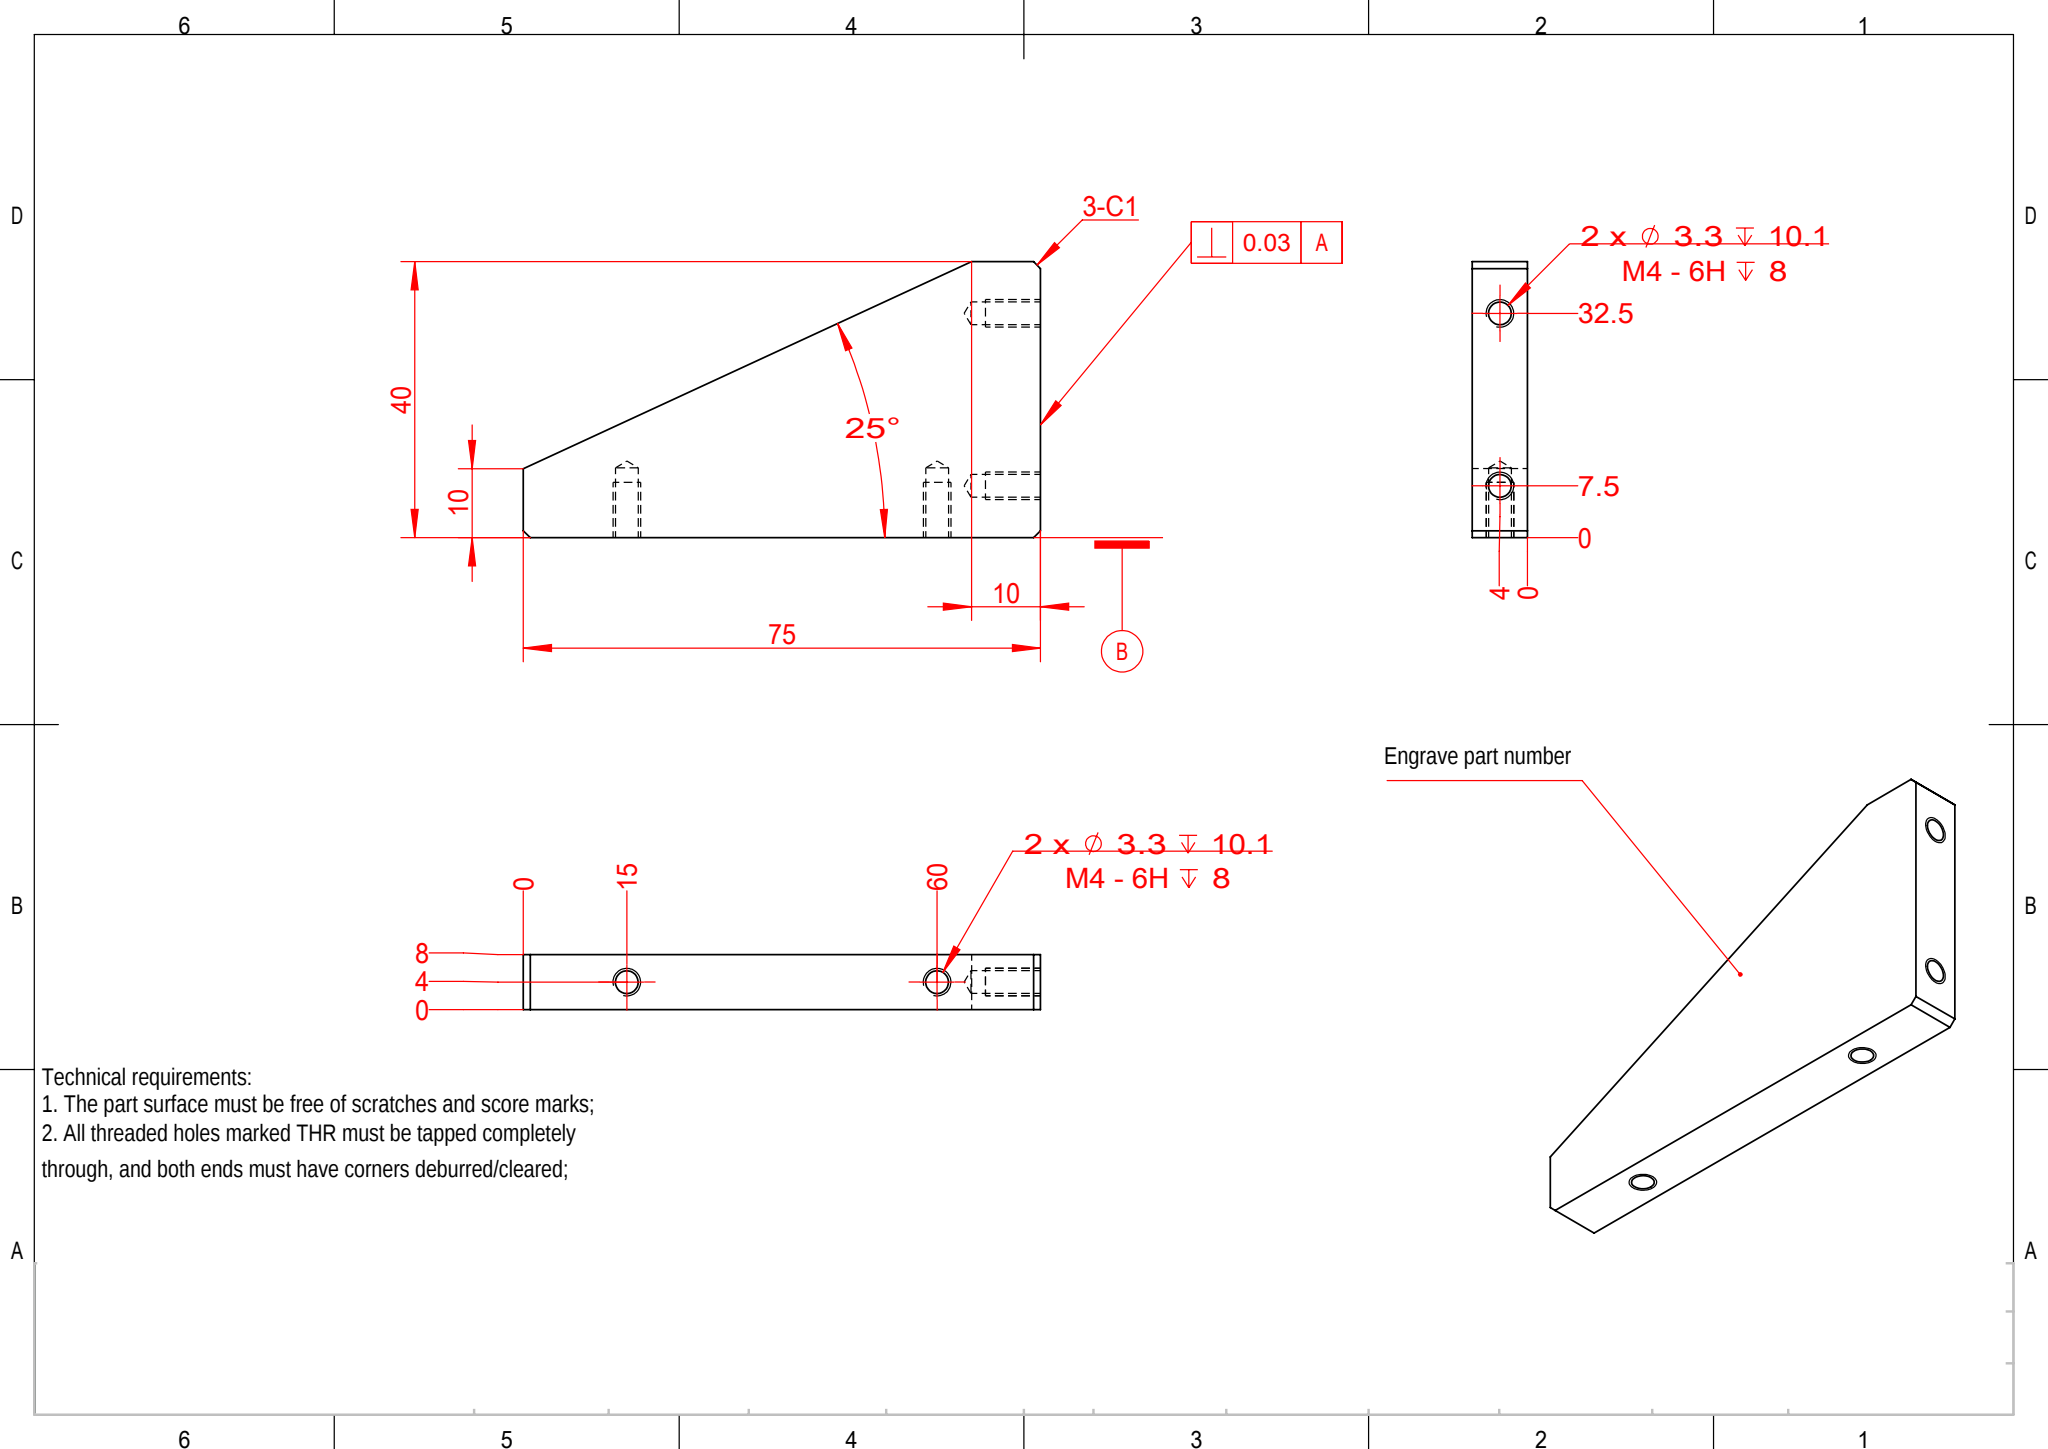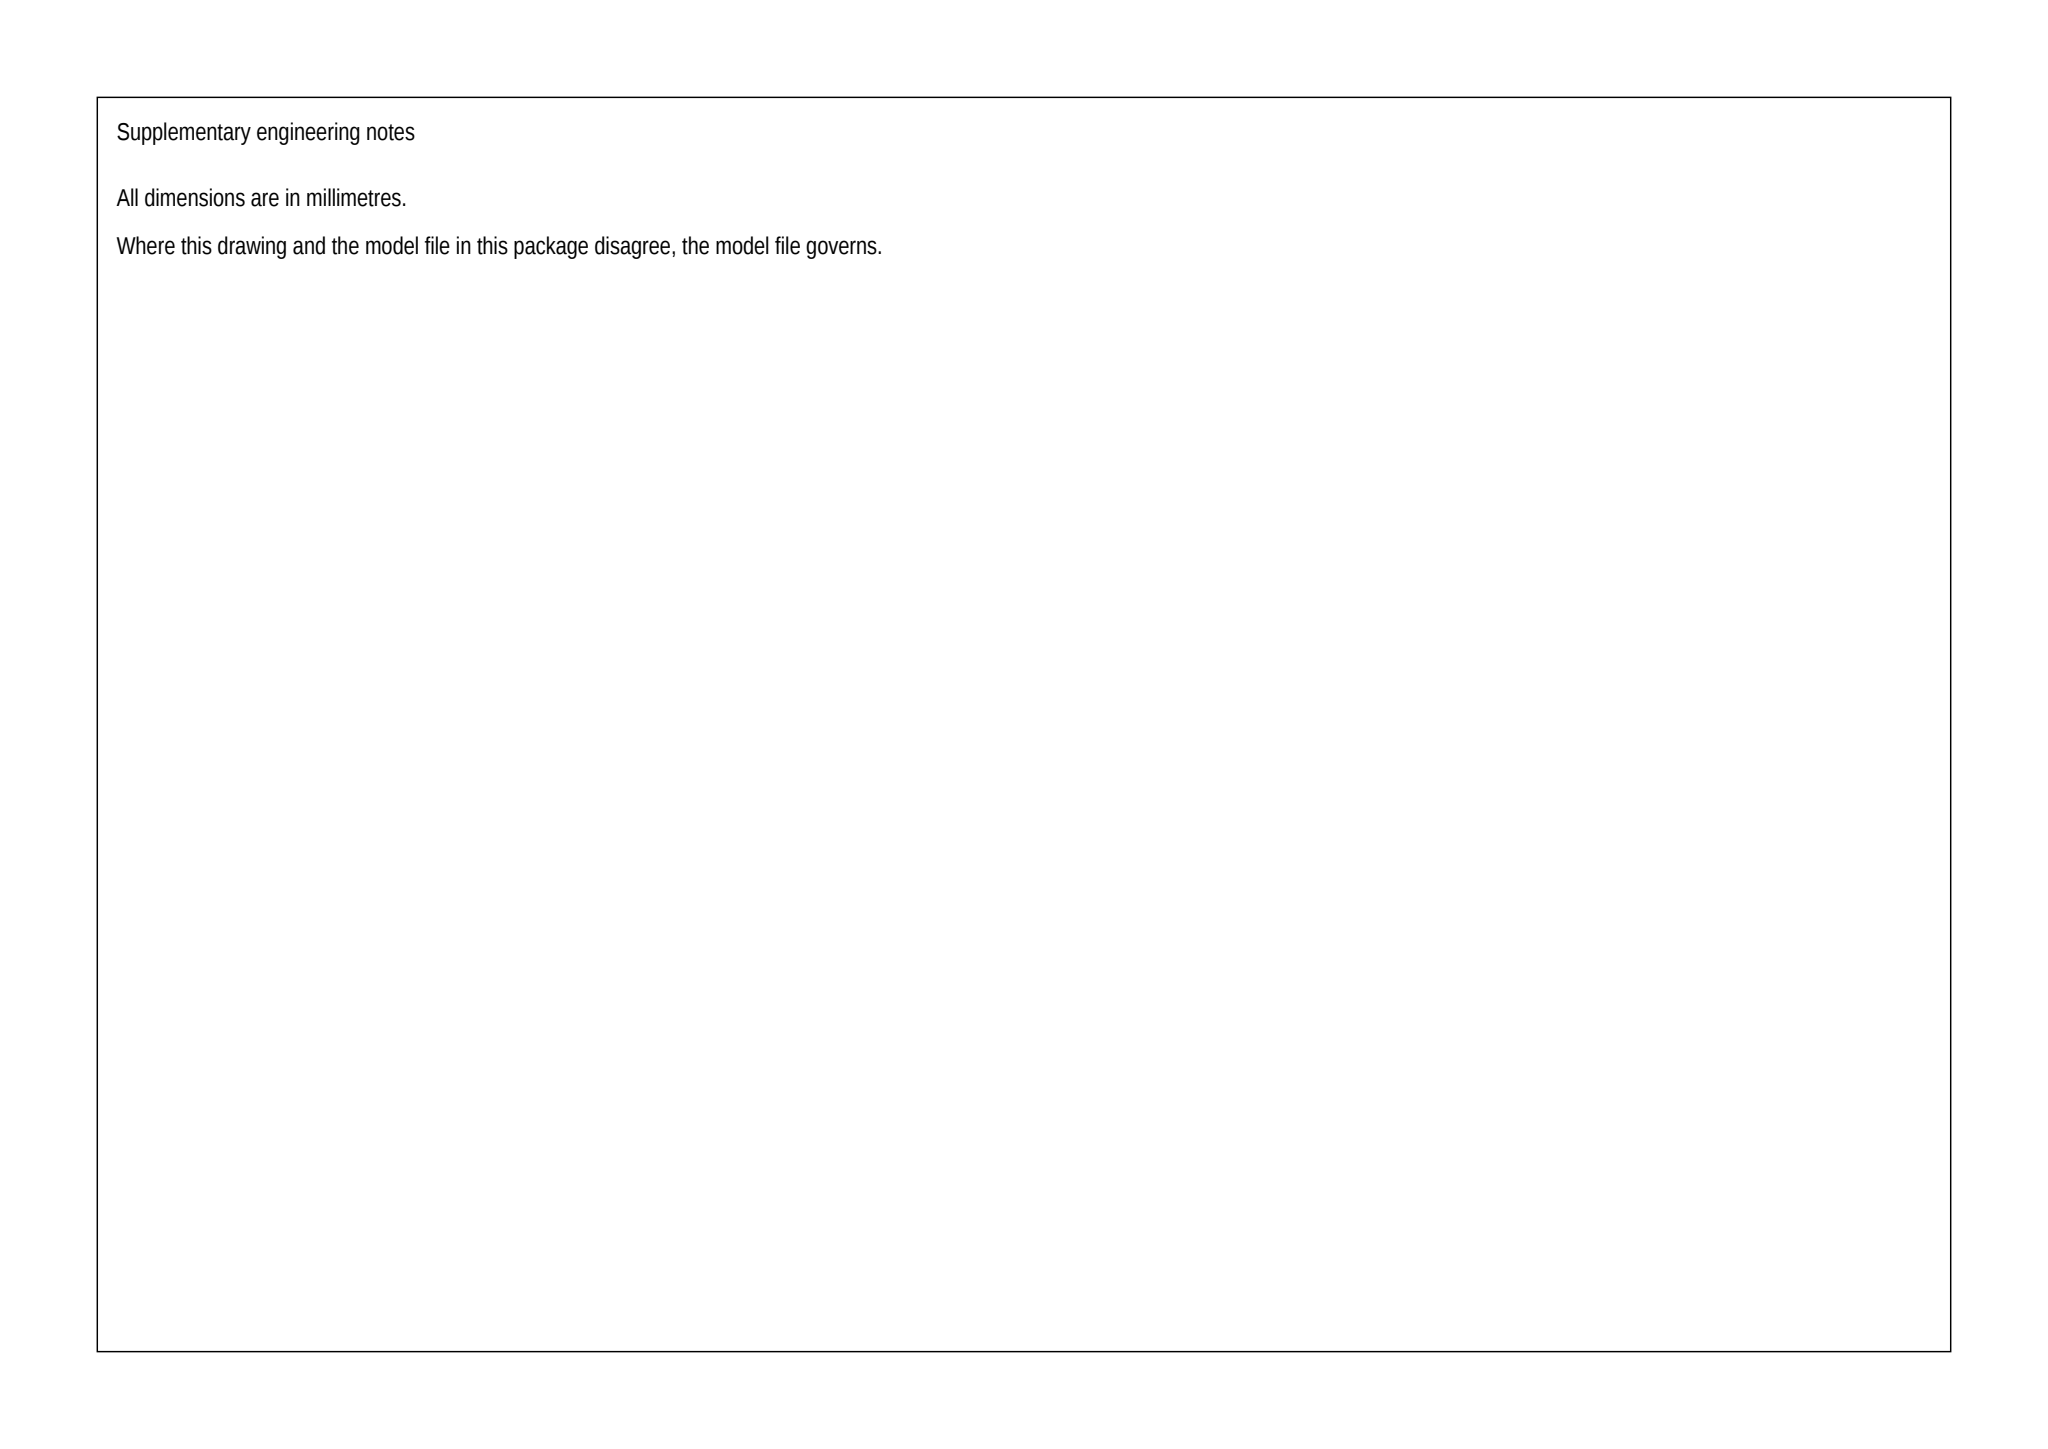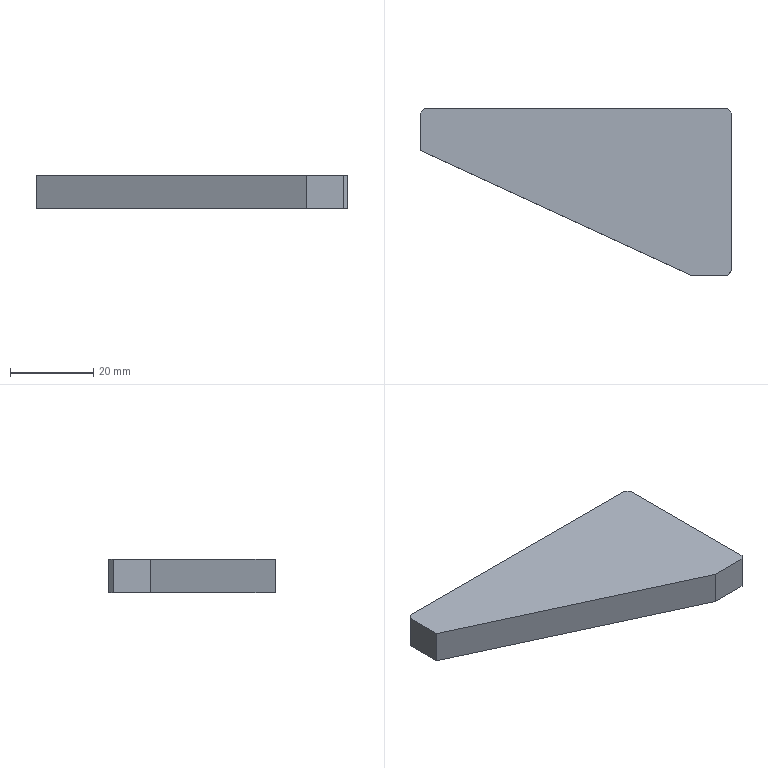Part | SolidWorks | mm | 1 solid | 26 faces | box 75 x 40 x 8 mm | volume 15831 mm3 | plane 10 | cylinder 8 | cone 8 | commonest cylinder face diameters 3.3 x8
build123d program:
from build123d import *

# Parameters (mm, degrees)
SKETCH1_W             = 75
SKETCH1_H             = 40
BOSS_EXTRUDE1_DEPTH   = 8
CUT_EXTRUDE1_DEPTH    = 44.246
M4_TAPPED_HOLE1_D     = 3.3
M4_TAPPED_HOLE1_DEPTH = 10.1
M4_TAPPED_HOLE1_TIP   = 0.9914
M4_TAPPED_HOLE2_D     = 3.3
M4_TAPPED_HOLE2_DEPTH = 10.1
M4_TAPPED_HOLE2_TIP   = 0.9914
CHAMFER1_SIZE         = 1


with BuildPart() as part:
    # Sketch1 → Boss-Extrude1 (new body)
    with BuildSketch(Plane.XY):
        Rectangle(SKETCH1_W, SKETCH1_H)
    extrude(amount=BOSS_EXTRUDE1_DEPTH)

    # Sketch2 → Cut-Extrude1 (cut, through all)
    with BuildSketch(Plane.XY.offset(8)):
        Polygon((-37.5, -20), (-37.5, 10), (27.5, -20), align=None)
    extrude(amount=-CUT_EXTRUDE1_DEPTH, mode=Mode.SUBTRACT)

    # M4 Tapped Hole1
    with Locations(Plane(origin=(0, 20, 0), x_dir=(1, 0, 0), z_dir=(0, 1, 0))):
        with Locations((22.5, -4), (-22.5, -4)):
            Hole(M4_TAPPED_HOLE1_D / 2, depth=M4_TAPPED_HOLE1_DEPTH)
            with Locations((0, 0, -(M4_TAPPED_HOLE1_DEPTH + M4_TAPPED_HOLE1_TIP / 2))):  # 118° drill point
                Cone(0, M4_TAPPED_HOLE1_D / 2, M4_TAPPED_HOLE1_TIP, mode=Mode.SUBTRACT)

    # M4 Tapped Hole2
    with Locations(Plane(origin=(37.5, 0, 0), x_dir=(0, 0, -1), z_dir=(1, 0, 0))):
        with Locations((-4, -12.5), (-4, 12.5)):
            Hole(M4_TAPPED_HOLE2_D / 2, depth=M4_TAPPED_HOLE2_DEPTH)
            with Locations((0, 0, -(M4_TAPPED_HOLE2_DEPTH + M4_TAPPED_HOLE2_TIP / 2))):  # 118° drill point
                Cone(0, M4_TAPPED_HOLE2_D / 2, M4_TAPPED_HOLE2_TIP, mode=Mode.SUBTRACT)

    # Chamfer1
    chamfer1_edges = [part.edges().sort_by_distance(p)[0] for p in [
        (37.5, -20, 4),
        (-37.5, 20, 4),
        (37.5, 20, 4),
    ]]
    chamfer(chamfer1_edges, length=CHAMFER1_SIZE)


solid = part.part
STEP:
#1=CARTESIAN_POINT('',(27.4,-12.5,5.65));
#2=VERTEX_POINT('',#1);
#3=CARTESIAN_POINT('',(27.4,-12.5,2.35));
#4=VERTEX_POINT('',#3);
#5=CARTESIAN_POINT('',(27.4,-12.5,4.));
#6=DIRECTION('',(1.,0.,0.));
#7=DIRECTION('',(0.,0.,-1.));
#8=AXIS2_PLACEMENT_3D('',#5,#6,#7);
#9=CIRCLE('',#8,1.65);
#10=EDGE_CURVE('',#2,#4,#9,.T.);
#11=ORIENTED_EDGE('',*,*,#10,.F.);
#12=CARTESIAN_POINT('',(37.5,-12.5,5.65));
#13=VERTEX_POINT('',#12);
#14=CARTESIAN_POINT('',(37.5,-12.5,5.65));
#15=DIRECTION('',(1.,0.,0.));
#16=VECTOR('',#15,1000.);
#17=LINE('',#14,#16);
#18=EDGE_CURVE('',#2,#13,#17,.T.);
#19=ORIENTED_EDGE('',*,*,#18,.T.);
#20=CARTESIAN_POINT('',(37.5,-12.5,2.35));
#21=VERTEX_POINT('',#20);
#22=CARTESIAN_POINT('',(37.5,-12.5,4.));
#23=DIRECTION('',(1.,0.,0.));
#24=DIRECTION('',(0.,0.,-1.));
#25=AXIS2_PLACEMENT_3D('',#22,#23,#24);
#26=CIRCLE('',#25,1.65);
#27=EDGE_CURVE('',#13,#21,#26,.T.);
#28=ORIENTED_EDGE('',*,*,#27,.T.);
#29=CARTESIAN_POINT('',(37.5,-12.5,2.35));
#30=DIRECTION('',(1.,0.,0.));
#31=VECTOR('',#30,1000.);
#32=LINE('',#29,#31);
#33=EDGE_CURVE('',#4,#21,#32,.T.);
#34=ORIENTED_EDGE('',*,*,#33,.F.);
#35=EDGE_LOOP('',(#11,#19,#28,#34));
#36=FACE_OUTER_BOUND('',#35,.T.);
#37=CARTESIAN_POINT('',(37.5,-12.5,4.));
#38=DIRECTION('',(1.,0.,0.));
#39=DIRECTION('',(0.,0.,-1.));
#40=AXIS2_PLACEMENT_3D('',#37,#38,#39);
#41=CYLINDRICAL_SURFACE('',#40,1.65);
#42=ADVANCED_FACE('',(#36),#41,.F.);
#43=CARTESIAN_POINT('',(26.409,-12.5,4.));
#44=VERTEX_POINT('',#43);
#45=CARTESIAN_POINT('',(27.4,-12.5,2.35));
#46=DIRECTION('',(0.515,0.,-0.8572));
#47=VECTOR('',#46,1000.);
#48=LINE('',#45,#47);
#49=EDGE_CURVE('',#44,#4,#48,.T.);
#50=ORIENTED_EDGE('',*,*,#49,.F.);
#51=CARTESIAN_POINT('',(27.4,-12.5,5.65));
#52=DIRECTION('',(0.515,0.,0.8572));
#53=VECTOR('',#52,1000.);
#54=LINE('',#51,#53);
#55=EDGE_CURVE('',#44,#2,#54,.T.);
#56=ORIENTED_EDGE('',*,*,#55,.T.);
#57=ORIENTED_EDGE('',*,*,#10,.T.);
#58=EDGE_LOOP('',(#50,#56,#57));
#59=FACE_OUTER_BOUND('',#58,.T.);
#60=CARTESIAN_POINT('',(27.4,-12.5,4.));
#61=DIRECTION('',(1.,0.,0.));
#62=DIRECTION('',(0.,0.,-1.));
#63=AXIS2_PLACEMENT_3D('',#60,#61,#62);
#64=CONICAL_SURFACE('',#63,1.65,1.03);
#65=ADVANCED_FACE('',(#59),#64,.F.);
#66=CARTESIAN_POINT('',(27.4,12.5,5.65));
#67=VERTEX_POINT('',#66);
#68=CARTESIAN_POINT('',(27.4,12.5,2.35));
#69=VERTEX_POINT('',#68);
#70=CARTESIAN_POINT('',(27.4,12.5,4.));
#71=DIRECTION('',(1.,0.,0.));
#72=DIRECTION('',(0.,0.,-1.));
#73=AXIS2_PLACEMENT_3D('',#70,#71,#72);
#74=CIRCLE('',#73,1.65);
#75=EDGE_CURVE('',#67,#69,#74,.T.);
#76=ORIENTED_EDGE('',*,*,#75,.F.);
#77=CARTESIAN_POINT('',(37.5,12.5,5.65));
#78=VERTEX_POINT('',#77);
#79=CARTESIAN_POINT('',(37.5,12.5,5.65));
#80=DIRECTION('',(1.,0.,0.));
#81=VECTOR('',#80,1000.);
#82=LINE('',#79,#81);
#83=EDGE_CURVE('',#67,#78,#82,.T.);
#84=ORIENTED_EDGE('',*,*,#83,.T.);
#85=CARTESIAN_POINT('',(37.5,12.5,2.35));
#86=VERTEX_POINT('',#85);
#87=CARTESIAN_POINT('',(37.5,12.5,4.));
#88=DIRECTION('',(1.,0.,0.));
#89=DIRECTION('',(0.,0.,-1.));
#90=AXIS2_PLACEMENT_3D('',#87,#88,#89);
#91=CIRCLE('',#90,1.65);
#92=EDGE_CURVE('',#78,#86,#91,.T.);
#93=ORIENTED_EDGE('',*,*,#92,.T.);
#94=CARTESIAN_POINT('',(37.5,12.5,2.35));
#95=DIRECTION('',(1.,0.,0.));
#96=VECTOR('',#95,1000.);
#97=LINE('',#94,#96);
#98=EDGE_CURVE('',#69,#86,#97,.T.);
#99=ORIENTED_EDGE('',*,*,#98,.F.);
#100=EDGE_LOOP('',(#76,#84,#93,#99));
#101=FACE_OUTER_BOUND('',#100,.T.);
#102=CARTESIAN_POINT('',(37.5,12.5,4.));
#103=DIRECTION('',(1.,0.,0.));
#104=DIRECTION('',(0.,0.,-1.));
#105=AXIS2_PLACEMENT_3D('',#102,#103,#104);
#106=CYLINDRICAL_SURFACE('',#105,1.65);
#107=ADVANCED_FACE('',(#101),#106,.F.);
#108=CARTESIAN_POINT('',(26.409,12.5,4.));
#109=VERTEX_POINT('',#108);
#110=CARTESIAN_POINT('',(27.4,12.5,2.35));
#111=DIRECTION('',(0.515,0.,-0.8572));
#112=VECTOR('',#111,1000.);
#113=LINE('',#110,#112);
#114=EDGE_CURVE('',#109,#69,#113,.T.);
#115=ORIENTED_EDGE('',*,*,#114,.F.);
#116=CARTESIAN_POINT('',(27.4,12.5,5.65));
#117=DIRECTION('',(0.515,0.,0.8572));
#118=VECTOR('',#117,1000.);
#119=LINE('',#116,#118);
#120=EDGE_CURVE('',#109,#67,#119,.T.);
#121=ORIENTED_EDGE('',*,*,#120,.T.);
#122=ORIENTED_EDGE('',*,*,#75,.T.);
#123=EDGE_LOOP('',(#115,#121,#122));
#124=FACE_OUTER_BOUND('',#123,.T.);
#125=CARTESIAN_POINT('',(27.4,12.5,4.));
#126=DIRECTION('',(1.,0.,0.));
#127=DIRECTION('',(0.,0.,-1.));
#128=AXIS2_PLACEMENT_3D('',#125,#126,#127);
#129=CONICAL_SURFACE('',#128,1.65,1.03);
#130=ADVANCED_FACE('',(#124),#129,.F.);
#131=CARTESIAN_POINT('',(22.5,9.9,2.35));
#132=VERTEX_POINT('',#131);
#133=CARTESIAN_POINT('',(22.5,9.9,5.65));
#134=VERTEX_POINT('',#133);
#135=CARTESIAN_POINT('',(22.5,9.9,4.));
#136=DIRECTION('',(0.,1.,0.));
#137=DIRECTION('',(0.,0.,1.));
#138=AXIS2_PLACEMENT_3D('',#135,#136,#137);
#139=CIRCLE('',#138,1.65);
#140=EDGE_CURVE('',#132,#134,#139,.T.);
#141=ORIENTED_EDGE('',*,*,#140,.F.);
#142=CARTESIAN_POINT('',(22.5,20.,2.35));
#143=VERTEX_POINT('',#142);
#144=CARTESIAN_POINT('',(22.5,20.,2.35));
#145=DIRECTION('',(0.,1.,0.));
#146=VECTOR('',#145,1000.);
#147=LINE('',#144,#146);
#148=EDGE_CURVE('',#132,#143,#147,.T.);
#149=ORIENTED_EDGE('',*,*,#148,.T.);
#150=CARTESIAN_POINT('',(22.5,20.,5.65));
#151=VERTEX_POINT('',#150);
#152=CARTESIAN_POINT('',(22.5,20.,4.));
#153=DIRECTION('',(0.,1.,0.));
#154=DIRECTION('',(0.,0.,1.));
#155=AXIS2_PLACEMENT_3D('',#152,#153,#154);
#156=CIRCLE('',#155,1.65);
#157=EDGE_CURVE('',#143,#151,#156,.T.);
#158=ORIENTED_EDGE('',*,*,#157,.T.);
#159=CARTESIAN_POINT('',(22.5,20.,5.65));
#160=DIRECTION('',(0.,1.,0.));
#161=VECTOR('',#160,1000.);
#162=LINE('',#159,#161);
#163=EDGE_CURVE('',#134,#151,#162,.T.);
#164=ORIENTED_EDGE('',*,*,#163,.F.);
#165=EDGE_LOOP('',(#141,#149,#158,#164));
#166=FACE_OUTER_BOUND('',#165,.T.);
#167=CARTESIAN_POINT('',(22.5,20.,4.));
#168=DIRECTION('',(0.,1.,0.));
#169=DIRECTION('',(0.,0.,1.));
#170=AXIS2_PLACEMENT_3D('',#167,#168,#169);
#171=CYLINDRICAL_SURFACE('',#170,1.65);
#172=ADVANCED_FACE('',(#166),#171,.F.);
#173=CARTESIAN_POINT('',(22.5,8.909,4.));
#174=VERTEX_POINT('',#173);
#175=CARTESIAN_POINT('',(22.5,9.9,5.65));
#176=DIRECTION('',(0.,0.515,0.8572));
#177=VECTOR('',#176,1000.);
#178=LINE('',#175,#177);
#179=EDGE_CURVE('',#174,#134,#178,.T.);
#180=ORIENTED_EDGE('',*,*,#179,.F.);
#181=CARTESIAN_POINT('',(22.5,9.9,2.35));
#182=DIRECTION('',(0.,0.515,-0.8572));
#183=VECTOR('',#182,1000.);
#184=LINE('',#181,#183);
#185=EDGE_CURVE('',#174,#132,#184,.T.);
#186=ORIENTED_EDGE('',*,*,#185,.T.);
#187=ORIENTED_EDGE('',*,*,#140,.T.);
#188=EDGE_LOOP('',(#180,#186,#187));
#189=FACE_OUTER_BOUND('',#188,.T.);
#190=CARTESIAN_POINT('',(22.5,9.9,4.));
#191=DIRECTION('',(0.,1.,0.));
#192=DIRECTION('',(0.,0.,1.));
#193=AXIS2_PLACEMENT_3D('',#190,#191,#192);
#194=CONICAL_SURFACE('',#193,1.65,1.03);
#195=ADVANCED_FACE('',(#189),#194,.F.);
#196=CARTESIAN_POINT('',(-22.5,9.9,2.35));
#197=VERTEX_POINT('',#196);
#198=CARTESIAN_POINT('',(-22.5,9.9,5.65));
#199=VERTEX_POINT('',#198);
#200=CARTESIAN_POINT('',(-22.5,9.9,4.));
#201=DIRECTION('',(0.,1.,0.));
#202=DIRECTION('',(0.,0.,1.));
#203=AXIS2_PLACEMENT_3D('',#200,#201,#202);
#204=CIRCLE('',#203,1.65);
#205=EDGE_CURVE('',#197,#199,#204,.T.);
#206=ORIENTED_EDGE('',*,*,#205,.F.);
#207=CARTESIAN_POINT('',(-22.5,20.,2.35));
#208=VERTEX_POINT('',#207);
#209=CARTESIAN_POINT('',(-22.5,20.,2.35));
#210=DIRECTION('',(0.,1.,0.));
#211=VECTOR('',#210,1000.);
#212=LINE('',#209,#211);
#213=EDGE_CURVE('',#197,#208,#212,.T.);
#214=ORIENTED_EDGE('',*,*,#213,.T.);
#215=CARTESIAN_POINT('',(-22.5,20.,5.65));
#216=VERTEX_POINT('',#215);
#217=CARTESIAN_POINT('',(-22.5,20.,4.));
#218=DIRECTION('',(0.,1.,0.));
#219=DIRECTION('',(0.,0.,1.));
#220=AXIS2_PLACEMENT_3D('',#217,#218,#219);
#221=CIRCLE('',#220,1.65);
#222=EDGE_CURVE('',#208,#216,#221,.T.);
#223=ORIENTED_EDGE('',*,*,#222,.T.);
#224=CARTESIAN_POINT('',(-22.5,20.,5.65));
#225=DIRECTION('',(0.,1.,0.));
#226=VECTOR('',#225,1000.);
#227=LINE('',#224,#226);
#228=EDGE_CURVE('',#199,#216,#227,.T.);
#229=ORIENTED_EDGE('',*,*,#228,.F.);
#230=EDGE_LOOP('',(#206,#214,#223,#229));
#231=FACE_OUTER_BOUND('',#230,.T.);
#232=CARTESIAN_POINT('',(-22.5,20.,4.));
#233=DIRECTION('',(0.,1.,0.));
#234=DIRECTION('',(0.,0.,1.));
#235=AXIS2_PLACEMENT_3D('',#232,#233,#234);
#236=CYLINDRICAL_SURFACE('',#235,1.65);
#237=ADVANCED_FACE('',(#231),#236,.F.);
#238=CARTESIAN_POINT('',(-22.5,8.909,4.));
#239=VERTEX_POINT('',#238);
#240=CARTESIAN_POINT('',(-22.5,9.9,5.65));
#241=DIRECTION('',(0.,0.515,0.8572));
#242=VECTOR('',#241,1000.);
#243=LINE('',#240,#242);
#244=EDGE_CURVE('',#239,#199,#243,.T.);
#245=ORIENTED_EDGE('',*,*,#244,.F.);
#246=CARTESIAN_POINT('',(-22.5,9.9,2.35));
#247=DIRECTION('',(0.,0.515,-0.8572));
#248=VECTOR('',#247,1000.);
#249=LINE('',#246,#248);
#250=EDGE_CURVE('',#239,#197,#249,.T.);
#251=ORIENTED_EDGE('',*,*,#250,.T.);
#252=ORIENTED_EDGE('',*,*,#205,.T.);
#253=EDGE_LOOP('',(#245,#251,#252));
#254=FACE_OUTER_BOUND('',#253,.T.);
#255=CARTESIAN_POINT('',(-22.5,9.9,4.));
#256=DIRECTION('',(0.,1.,0.));
#257=DIRECTION('',(0.,0.,1.));
#258=AXIS2_PLACEMENT_3D('',#255,#256,#257);
#259=CONICAL_SURFACE('',#258,1.65,1.03);
#260=ADVANCED_FACE('',(#254),#259,.F.);
#261=CARTESIAN_POINT('',(22.5,20.,4.));
#262=DIRECTION('',(0.,1.,0.));
#263=DIRECTION('',(0.,0.,1.));
#264=AXIS2_PLACEMENT_3D('',#261,#262,#263);
#265=CIRCLE('',#264,1.65);
#266=EDGE_CURVE('',#151,#143,#265,.T.);
#267=ORIENTED_EDGE('',*,*,#266,.F.);
#268=ORIENTED_EDGE('',*,*,#157,.F.);
#269=EDGE_LOOP('',(#267,#268));
#270=FACE_BOUND('',#269,.T.);
#271=CARTESIAN_POINT('',(36.5,20.,0.));
#272=VERTEX_POINT('',#271);
#273=CARTESIAN_POINT('',(-36.5,20.,0.));
#274=VERTEX_POINT('',#273);
#275=CARTESIAN_POINT('',(-37.5,20.,0.));
#276=DIRECTION('',(-1.,0.,0.));
#277=VECTOR('',#276,1000.);
#278=LINE('',#275,#277);
#279=EDGE_CURVE('',#272,#274,#278,.T.);
#280=ORIENTED_EDGE('',*,*,#279,.T.);
#281=CARTESIAN_POINT('',(-36.5,20.,8.));
#282=VERTEX_POINT('',#281);
#283=CARTESIAN_POINT('',(-36.5,20.,8.));
#284=DIRECTION('',(0.,0.,1.));
#285=VECTOR('',#284,1000.);
#286=LINE('',#283,#285);
#287=EDGE_CURVE('',#274,#282,#286,.T.);
#288=ORIENTED_EDGE('',*,*,#287,.T.);
#289=CARTESIAN_POINT('',(36.5,20.,8.));
#290=VERTEX_POINT('',#289);
#291=CARTESIAN_POINT('',(-37.5,20.,8.));
#292=DIRECTION('',(-1.,0.,0.));
#293=VECTOR('',#292,1000.);
#294=LINE('',#291,#293);
#295=EDGE_CURVE('',#290,#282,#294,.T.);
#296=ORIENTED_EDGE('',*,*,#295,.F.);
#297=CARTESIAN_POINT('',(36.5,20.,8.));
#298=DIRECTION('',(0.,0.,-1.));
#299=VECTOR('',#298,1000.);
#300=LINE('',#297,#299);
#301=EDGE_CURVE('',#290,#272,#300,.T.);
#302=ORIENTED_EDGE('',*,*,#301,.T.);
#303=EDGE_LOOP('',(#280,#288,#296,#302));
#304=FACE_OUTER_BOUND('',#303,.T.);
#305=CARTESIAN_POINT('',(-22.5,20.,4.));
#306=DIRECTION('',(0.,1.,0.));
#307=DIRECTION('',(0.,0.,1.));
#308=AXIS2_PLACEMENT_3D('',#305,#306,#307);
#309=CIRCLE('',#308,1.65);
#310=EDGE_CURVE('',#216,#208,#309,.T.);
#311=ORIENTED_EDGE('',*,*,#310,.F.);
#312=ORIENTED_EDGE('',*,*,#222,.F.);
#313=EDGE_LOOP('',(#311,#312));
#314=FACE_BOUND('',#313,.T.);
#315=CARTESIAN_POINT('',(-37.5,20.,8.));
#316=DIRECTION('',(0.,-1.,0.));
#317=DIRECTION('',(0.,0.,-1.));
#318=AXIS2_PLACEMENT_3D('',#315,#316,#317);
#319=PLANE('',#318);
#320=ADVANCED_FACE('',(#270,#304,#314),#319,.F.);
#321=CARTESIAN_POINT('',(37.5,-12.5,4.));
#322=DIRECTION('',(1.,0.,0.));
#323=DIRECTION('',(0.,0.,-1.));
#324=AXIS2_PLACEMENT_3D('',#321,#322,#323);
#325=CIRCLE('',#324,1.65);
#326=EDGE_CURVE('',#21,#13,#325,.T.);
#327=ORIENTED_EDGE('',*,*,#326,.F.);
#328=ORIENTED_EDGE('',*,*,#27,.F.);
#329=EDGE_LOOP('',(#327,#328));
#330=FACE_BOUND('',#329,.T.);
#331=CARTESIAN_POINT('',(37.5,12.5,4.));
#332=DIRECTION('',(1.,0.,0.));
#333=DIRECTION('',(0.,0.,-1.));
#334=AXIS2_PLACEMENT_3D('',#331,#332,#333);
#335=CIRCLE('',#334,1.65);
#336=EDGE_CURVE('',#86,#78,#335,.T.);
#337=ORIENTED_EDGE('',*,*,#336,.F.);
#338=ORIENTED_EDGE('',*,*,#92,.F.);
#339=EDGE_LOOP('',(#337,#338));
#340=FACE_BOUND('',#339,.T.);
#341=CARTESIAN_POINT('',(37.5,-19.,8.));
#342=VERTEX_POINT('',#341);
#343=CARTESIAN_POINT('',(37.5,19.,8.));
#344=VERTEX_POINT('',#343);
#345=CARTESIAN_POINT('',(37.5,20.,8.));
#346=DIRECTION('',(-0.,1.,0.));
#347=VECTOR('',#346,1000.);
#348=LINE('',#345,#347);
#349=EDGE_CURVE('',#342,#344,#348,.T.);
#350=ORIENTED_EDGE('',*,*,#349,.F.);
#351=CARTESIAN_POINT('',(37.5,-19.,0.));
#352=VERTEX_POINT('',#351);
#353=CARTESIAN_POINT('',(37.5,-19.,8.));
#354=DIRECTION('',(0.,0.,-1.));
#355=VECTOR('',#354,1000.);
#356=LINE('',#353,#355);
#357=EDGE_CURVE('',#342,#352,#356,.T.);
#358=ORIENTED_EDGE('',*,*,#357,.T.);
#359=CARTESIAN_POINT('',(37.5,19.,0.));
#360=VERTEX_POINT('',#359);
#361=CARTESIAN_POINT('',(37.5,20.,0.));
#362=DIRECTION('',(-0.,1.,0.));
#363=VECTOR('',#362,1000.);
#364=LINE('',#361,#363);
#365=EDGE_CURVE('',#352,#360,#364,.T.);
#366=ORIENTED_EDGE('',*,*,#365,.T.);
#367=CARTESIAN_POINT('',(37.5,19.,8.));
#368=DIRECTION('',(0.,0.,1.));
#369=VECTOR('',#368,1000.);
#370=LINE('',#367,#369);
#371=EDGE_CURVE('',#360,#344,#370,.T.);
#372=ORIENTED_EDGE('',*,*,#371,.T.);
#373=EDGE_LOOP('',(#350,#358,#366,#372));
#374=FACE_OUTER_BOUND('',#373,.T.);
#375=CARTESIAN_POINT('',(37.5,20.,8.));
#376=DIRECTION('',(-1.,-0.,0.));
#377=DIRECTION('',(0.,-1.,0.));
#378=AXIS2_PLACEMENT_3D('',#375,#376,#377);
#379=PLANE('',#378);
#380=ADVANCED_FACE('',(#330,#340,#374),#379,.F.);
#381=CARTESIAN_POINT('',(-37.5,19.,8.));
#382=VERTEX_POINT('',#381);
#383=CARTESIAN_POINT('',(-37.5,10.,8.));
#384=VERTEX_POINT('',#383);
#385=CARTESIAN_POINT('',(-37.5,20.,8.));
#386=DIRECTION('',(0.,-1.,0.));
#387=VECTOR('',#386,1000.);
#388=LINE('',#385,#387);
#389=EDGE_CURVE('',#382,#384,#388,.T.);
#390=ORIENTED_EDGE('',*,*,#389,.F.);
#391=CARTESIAN_POINT('',(-37.5,19.,0.));
#392=VERTEX_POINT('',#391);
#393=CARTESIAN_POINT('',(-37.5,19.,8.));
#394=DIRECTION('',(0.,0.,-1.));
#395=VECTOR('',#394,1000.);
#396=LINE('',#393,#395);
#397=EDGE_CURVE('',#382,#392,#396,.T.);
#398=ORIENTED_EDGE('',*,*,#397,.T.);
#399=CARTESIAN_POINT('',(-37.5,10.,0.));
#400=VERTEX_POINT('',#399);
#401=CARTESIAN_POINT('',(-37.5,20.,0.));
#402=DIRECTION('',(0.,-1.,0.));
#403=VECTOR('',#402,1000.);
#404=LINE('',#401,#403);
#405=EDGE_CURVE('',#392,#400,#404,.T.);
#406=ORIENTED_EDGE('',*,*,#405,.T.);
#407=CARTESIAN_POINT('',(-37.5,10.,0.));
#408=DIRECTION('',(0.,0.,1.));
#409=VECTOR('',#408,1000.);
#410=LINE('',#407,#409);
#411=EDGE_CURVE('',#400,#384,#410,.T.);
#412=ORIENTED_EDGE('',*,*,#411,.T.);
#413=EDGE_LOOP('',(#390,#398,#406,#412));
#414=FACE_OUTER_BOUND('',#413,.T.);
#415=CARTESIAN_POINT('',(-37.5,20.,8.));
#416=DIRECTION('',(1.,0.,0.));
#417=DIRECTION('',(-0.,1.,0.));
#418=AXIS2_PLACEMENT_3D('',#415,#416,#417);
#419=PLANE('',#418);
#420=ADVANCED_FACE('',(#414),#419,.F.);
#421=CARTESIAN_POINT('',(27.5,-20.,0.));
#422=VERTEX_POINT('',#421);
#423=CARTESIAN_POINT('',(36.5,-20.,0.));
#424=VERTEX_POINT('',#423);
#425=CARTESIAN_POINT('',(-37.5,-20.,0.));
#426=DIRECTION('',(1.,0.,0.));
#427=VECTOR('',#426,1000.);
#428=LINE('',#425,#427);
#429=EDGE_CURVE('',#422,#424,#428,.T.);
#430=ORIENTED_EDGE('',*,*,#429,.T.);
#431=CARTESIAN_POINT('',(36.5,-20.,8.));
#432=VERTEX_POINT('',#431);
#433=CARTESIAN_POINT('',(36.5,-20.,8.));
#434=DIRECTION('',(0.,0.,1.));
#435=VECTOR('',#434,1000.);
#436=LINE('',#433,#435);
#437=EDGE_CURVE('',#424,#432,#436,.T.);
#438=ORIENTED_EDGE('',*,*,#437,.T.);
#439=CARTESIAN_POINT('',(27.5,-20.,8.));
#440=VERTEX_POINT('',#439);
#441=CARTESIAN_POINT('',(-37.5,-20.,8.));
#442=DIRECTION('',(1.,0.,0.));
#443=VECTOR('',#442,1000.);
#444=LINE('',#441,#443);
#445=EDGE_CURVE('',#440,#432,#444,.T.);
#446=ORIENTED_EDGE('',*,*,#445,.F.);
#447=CARTESIAN_POINT('',(27.5,-20.,0.));
#448=DIRECTION('',(0.,0.,1.));
#449=VECTOR('',#448,1000.);
#450=LINE('',#447,#449);
#451=EDGE_CURVE('',#422,#440,#450,.T.);
#452=ORIENTED_EDGE('',*,*,#451,.F.);
#453=EDGE_LOOP('',(#430,#438,#446,#452));
#454=FACE_OUTER_BOUND('',#453,.T.);
#455=CARTESIAN_POINT('',(-37.5,-20.,8.));
#456=DIRECTION('',(0.,1.,0.));
#457=DIRECTION('',(0.,0.,1.));
#458=AXIS2_PLACEMENT_3D('',#455,#456,#457);
#459=PLANE('',#458);
#460=ADVANCED_FACE('',(#454),#459,.F.);
#461=ORIENTED_EDGE('',*,*,#445,.T.);
#462=CARTESIAN_POINT('',(28.25,-28.25,8.));
#463=DIRECTION('',(0.7071,0.7071,0.));
#464=VECTOR('',#463,1000.);
#465=LINE('',#462,#464);
#466=EDGE_CURVE('',#432,#342,#465,.T.);
#467=ORIENTED_EDGE('',*,*,#466,.T.);
#468=ORIENTED_EDGE('',*,*,#349,.T.);
#469=CARTESIAN_POINT('',(28.25,28.25,8.));
#470=DIRECTION('',(-0.7071,0.7071,0.));
#471=VECTOR('',#470,1000.);
#472=LINE('',#469,#471);
#473=EDGE_CURVE('',#344,#290,#472,.T.);
#474=ORIENTED_EDGE('',*,*,#473,.T.);
#475=ORIENTED_EDGE('',*,*,#295,.T.);
#476=CARTESIAN_POINT('',(-28.25,28.25,8.));
#477=DIRECTION('',(-0.7071,-0.7071,0.));
#478=VECTOR('',#477,1000.);
#479=LINE('',#476,#478);
#480=EDGE_CURVE('',#282,#382,#479,.T.);
#481=ORIENTED_EDGE('',*,*,#480,.T.);
#482=ORIENTED_EDGE('',*,*,#389,.T.);
#483=CARTESIAN_POINT('',(-37.5,10.,8.));
#484=DIRECTION('',(-0.908,0.4191,0.));
#485=VECTOR('',#484,1000.);
#486=LINE('',#483,#485);
#487=EDGE_CURVE('',#440,#384,#486,.T.);
#488=ORIENTED_EDGE('',*,*,#487,.F.);
#489=EDGE_LOOP('',(#461,#467,#468,#474,#475,#481,#482,#488));
#490=FACE_OUTER_BOUND('',#489,.T.);
#491=CARTESIAN_POINT('',(0.,0.,8.));
#492=DIRECTION('',(0.,0.,1.));
#493=DIRECTION('',(1.,0.,0.));
#494=AXIS2_PLACEMENT_3D('',#491,#492,#493);
#495=PLANE('',#494);
#496=ADVANCED_FACE('',(#490),#495,.T.);
#497=ORIENTED_EDGE('',*,*,#365,.F.);
#498=CARTESIAN_POINT('',(37.5,-19.,0.));
#499=DIRECTION('',(-0.7071,-0.7071,0.));
#500=VECTOR('',#499,1000.);
#501=LINE('',#498,#500);
#502=EDGE_CURVE('',#352,#424,#501,.T.);
#503=ORIENTED_EDGE('',*,*,#502,.T.);
#504=ORIENTED_EDGE('',*,*,#429,.F.);
#505=CARTESIAN_POINT('',(-37.5,10.,0.));
#506=DIRECTION('',(-0.908,0.4191,0.));
#507=VECTOR('',#506,1000.);
#508=LINE('',#505,#507);
#509=EDGE_CURVE('',#422,#400,#508,.T.);
#510=ORIENTED_EDGE('',*,*,#509,.T.);
#511=ORIENTED_EDGE('',*,*,#405,.F.);
#512=CARTESIAN_POINT('',(-37.5,19.,0.));
#513=DIRECTION('',(0.7071,0.7071,0.));
#514=VECTOR('',#513,1000.);
#515=LINE('',#512,#514);
#516=EDGE_CURVE('',#392,#274,#515,.T.);
#517=ORIENTED_EDGE('',*,*,#516,.T.);
#518=ORIENTED_EDGE('',*,*,#279,.F.);
#519=CARTESIAN_POINT('',(36.5,20.,0.));
#520=DIRECTION('',(0.7071,-0.7071,0.));
#521=VECTOR('',#520,1000.);
#522=LINE('',#519,#521);
#523=EDGE_CURVE('',#272,#360,#522,.T.);
#524=ORIENTED_EDGE('',*,*,#523,.T.);
#525=EDGE_LOOP('',(#497,#503,#504,#510,#511,#517,#518,#524));
#526=FACE_OUTER_BOUND('',#525,.T.);
#527=CARTESIAN_POINT('',(0.,0.,0.));
#528=DIRECTION('',(0.,0.,1.));
#529=DIRECTION('',(1.,0.,0.));
#530=AXIS2_PLACEMENT_3D('',#527,#528,#529);
#531=PLANE('',#530);
#532=ADVANCED_FACE('',(#526),#531,.F.);
#533=ORIENTED_EDGE('',*,*,#487,.T.);
#534=ORIENTED_EDGE('',*,*,#411,.F.);
#535=ORIENTED_EDGE('',*,*,#509,.F.);
#536=ORIENTED_EDGE('',*,*,#451,.T.);
#537=EDGE_LOOP('',(#533,#534,#535,#536));
#538=FACE_OUTER_BOUND('',#537,.T.);
#539=CARTESIAN_POINT('',(-37.5,10.,0.));
#540=DIRECTION('',(0.4191,0.908,0.));
#541=DIRECTION('',(-0.908,0.4191,0.));
#542=AXIS2_PLACEMENT_3D('',#539,#540,#541);
#543=PLANE('',#542);
#544=ADVANCED_FACE('',(#538),#543,.F.);
#545=ORIENTED_EDGE('',*,*,#250,.F.);
#546=ORIENTED_EDGE('',*,*,#244,.T.);
#547=CARTESIAN_POINT('',(-22.5,9.9,4.));
#548=DIRECTION('',(0.,1.,0.));
#549=DIRECTION('',(0.,0.,1.));
#550=AXIS2_PLACEMENT_3D('',#547,#548,#549);
#551=CIRCLE('',#550,1.65);
#552=EDGE_CURVE('',#199,#197,#551,.T.);
#553=ORIENTED_EDGE('',*,*,#552,.T.);
#554=EDGE_LOOP('',(#545,#546,#553));
#555=FACE_OUTER_BOUND('',#554,.T.);
#556=CARTESIAN_POINT('',(-22.5,9.9,4.));
#557=DIRECTION('',(0.,1.,0.));
#558=DIRECTION('',(0.,0.,1.));
#559=AXIS2_PLACEMENT_3D('',#556,#557,#558);
#560=CONICAL_SURFACE('',#559,1.65,1.03);
#561=ADVANCED_FACE('',(#555),#560,.F.);
#562=ORIENTED_EDGE('',*,*,#213,.F.);
#563=ORIENTED_EDGE('',*,*,#552,.F.);
#564=ORIENTED_EDGE('',*,*,#228,.T.);
#565=ORIENTED_EDGE('',*,*,#310,.T.);
#566=EDGE_LOOP('',(#562,#563,#564,#565));
#567=FACE_OUTER_BOUND('',#566,.T.);
#568=CARTESIAN_POINT('',(-22.5,20.,4.));
#569=DIRECTION('',(0.,1.,0.));
#570=DIRECTION('',(0.,0.,1.));
#571=AXIS2_PLACEMENT_3D('',#568,#569,#570);
#572=CYLINDRICAL_SURFACE('',#571,1.65);
#573=ADVANCED_FACE('',(#567),#572,.F.);
#574=ORIENTED_EDGE('',*,*,#185,.F.);
#575=ORIENTED_EDGE('',*,*,#179,.T.);
#576=CARTESIAN_POINT('',(22.5,9.9,4.));
#577=DIRECTION('',(0.,1.,0.));
#578=DIRECTION('',(0.,0.,1.));
#579=AXIS2_PLACEMENT_3D('',#576,#577,#578);
#580=CIRCLE('',#579,1.65);
#581=EDGE_CURVE('',#134,#132,#580,.T.);
#582=ORIENTED_EDGE('',*,*,#581,.T.);
#583=EDGE_LOOP('',(#574,#575,#582));
#584=FACE_OUTER_BOUND('',#583,.T.);
#585=CARTESIAN_POINT('',(22.5,9.9,4.));
#586=DIRECTION('',(0.,1.,0.));
#587=DIRECTION('',(0.,0.,1.));
#588=AXIS2_PLACEMENT_3D('',#585,#586,#587);
#589=CONICAL_SURFACE('',#588,1.65,1.03);
#590=ADVANCED_FACE('',(#584),#589,.F.);
#591=ORIENTED_EDGE('',*,*,#148,.F.);
#592=ORIENTED_EDGE('',*,*,#581,.F.);
#593=ORIENTED_EDGE('',*,*,#163,.T.);
#594=ORIENTED_EDGE('',*,*,#266,.T.);
#595=EDGE_LOOP('',(#591,#592,#593,#594));
#596=FACE_OUTER_BOUND('',#595,.T.);
#597=CARTESIAN_POINT('',(22.5,20.,4.));
#598=DIRECTION('',(0.,1.,0.));
#599=DIRECTION('',(0.,0.,1.));
#600=AXIS2_PLACEMENT_3D('',#597,#598,#599);
#601=CYLINDRICAL_SURFACE('',#600,1.65);
#602=ADVANCED_FACE('',(#596),#601,.F.);
#603=ORIENTED_EDGE('',*,*,#120,.F.);
#604=ORIENTED_EDGE('',*,*,#114,.T.);
#605=CARTESIAN_POINT('',(27.4,12.5,4.));
#606=DIRECTION('',(1.,0.,0.));
#607=DIRECTION('',(0.,0.,-1.));
#608=AXIS2_PLACEMENT_3D('',#605,#606,#607);
#609=CIRCLE('',#608,1.65);
#610=EDGE_CURVE('',#69,#67,#609,.T.);
#611=ORIENTED_EDGE('',*,*,#610,.T.);
#612=EDGE_LOOP('',(#603,#604,#611));
#613=FACE_OUTER_BOUND('',#612,.T.);
#614=CARTESIAN_POINT('',(27.4,12.5,4.));
#615=DIRECTION('',(1.,0.,0.));
#616=DIRECTION('',(0.,0.,-1.));
#617=AXIS2_PLACEMENT_3D('',#614,#615,#616);
#618=CONICAL_SURFACE('',#617,1.65,1.03);
#619=ADVANCED_FACE('',(#613),#618,.F.);
#620=ORIENTED_EDGE('',*,*,#83,.F.);
#621=ORIENTED_EDGE('',*,*,#610,.F.);
#622=ORIENTED_EDGE('',*,*,#98,.T.);
#623=ORIENTED_EDGE('',*,*,#336,.T.);
#624=EDGE_LOOP('',(#620,#621,#622,#623));
#625=FACE_OUTER_BOUND('',#624,.T.);
#626=CARTESIAN_POINT('',(37.5,12.5,4.));
#627=DIRECTION('',(1.,0.,0.));
#628=DIRECTION('',(0.,0.,-1.));
#629=AXIS2_PLACEMENT_3D('',#626,#627,#628);
#630=CYLINDRICAL_SURFACE('',#629,1.65);
#631=ADVANCED_FACE('',(#625),#630,.F.);
#632=ORIENTED_EDGE('',*,*,#55,.F.);
#633=ORIENTED_EDGE('',*,*,#49,.T.);
#634=CARTESIAN_POINT('',(27.4,-12.5,4.));
#635=DIRECTION('',(1.,0.,0.));
#636=DIRECTION('',(0.,0.,-1.));
#637=AXIS2_PLACEMENT_3D('',#634,#635,#636);
#638=CIRCLE('',#637,1.65);
#639=EDGE_CURVE('',#4,#2,#638,.T.);
#640=ORIENTED_EDGE('',*,*,#639,.T.);
#641=EDGE_LOOP('',(#632,#633,#640));
#642=FACE_OUTER_BOUND('',#641,.T.);
#643=CARTESIAN_POINT('',(27.4,-12.5,4.));
#644=DIRECTION('',(1.,0.,0.));
#645=DIRECTION('',(0.,0.,-1.));
#646=AXIS2_PLACEMENT_3D('',#643,#644,#645);
#647=CONICAL_SURFACE('',#646,1.65,1.03);
#648=ADVANCED_FACE('',(#642),#647,.F.);
#649=ORIENTED_EDGE('',*,*,#18,.F.);
#650=ORIENTED_EDGE('',*,*,#639,.F.);
#651=ORIENTED_EDGE('',*,*,#33,.T.);
#652=ORIENTED_EDGE('',*,*,#326,.T.);
#653=EDGE_LOOP('',(#649,#650,#651,#652));
#654=FACE_OUTER_BOUND('',#653,.T.);
#655=CARTESIAN_POINT('',(37.5,-12.5,4.));
#656=DIRECTION('',(1.,0.,0.));
#657=DIRECTION('',(0.,0.,-1.));
#658=AXIS2_PLACEMENT_3D('',#655,#656,#657);
#659=CYLINDRICAL_SURFACE('',#658,1.65);
#660=ADVANCED_FACE('',(#654),#659,.F.);
#661=ORIENTED_EDGE('',*,*,#466,.F.);
#662=ORIENTED_EDGE('',*,*,#437,.F.);
#663=ORIENTED_EDGE('',*,*,#502,.F.);
#664=ORIENTED_EDGE('',*,*,#357,.F.);
#665=EDGE_LOOP('',(#661,#662,#663,#664));
#666=FACE_OUTER_BOUND('',#665,.T.);
#667=CARTESIAN_POINT('',(37.5,-19.,8.));
#668=DIRECTION('',(-0.7071,0.7071,0.));
#669=DIRECTION('',(0.,0.,-1.));
#670=AXIS2_PLACEMENT_3D('',#667,#668,#669);
#671=PLANE('',#670);
#672=ADVANCED_FACE('',(#666),#671,.F.);
#673=ORIENTED_EDGE('',*,*,#480,.F.);
#674=ORIENTED_EDGE('',*,*,#287,.F.);
#675=ORIENTED_EDGE('',*,*,#516,.F.);
#676=ORIENTED_EDGE('',*,*,#397,.F.);
#677=EDGE_LOOP('',(#673,#674,#675,#676));
#678=FACE_OUTER_BOUND('',#677,.T.);
#679=CARTESIAN_POINT('',(-37.5,19.,8.));
#680=DIRECTION('',(0.7071,-0.7071,0.));
#681=DIRECTION('',(0.,0.,-1.));
#682=AXIS2_PLACEMENT_3D('',#679,#680,#681);
#683=PLANE('',#682);
#684=ADVANCED_FACE('',(#678),#683,.F.);
#685=ORIENTED_EDGE('',*,*,#473,.F.);
#686=ORIENTED_EDGE('',*,*,#371,.F.);
#687=ORIENTED_EDGE('',*,*,#523,.F.);
#688=ORIENTED_EDGE('',*,*,#301,.F.);
#689=EDGE_LOOP('',(#685,#686,#687,#688));
#690=FACE_OUTER_BOUND('',#689,.T.);
#691=CARTESIAN_POINT('',(36.5,20.,8.));
#692=DIRECTION('',(-0.7071,-0.7071,0.));
#693=DIRECTION('',(0.,0.,-1.));
#694=AXIS2_PLACEMENT_3D('',#691,#692,#693);
#695=PLANE('',#694);
#696=ADVANCED_FACE('',(#690),#695,.F.);
#697=CLOSED_SHELL('',(#42,#65,#107,#130,#172,#195,#237,#260,#320,#380,#420,#460,#496,#532,#544,#561,#573,#590,#602,#619,#631,#648,#660,#672,#684,#696));
#698=MANIFOLD_SOLID_BREP('',#697);
#699=CARTESIAN_POINT('',(0.,0.,0.));
#700=DIRECTION('',(0.,0.,1.));
#701=DIRECTION('',(1.,0.,0.));
#702=AXIS2_PLACEMENT_3D('',#699,#700,#701);
#703=(LENGTH_UNIT()NAMED_UNIT(*)SI_UNIT(.MILLI.,.METRE.));
#704=UNCERTAINTY_MEASURE_WITH_UNIT(LENGTH_MEASURE(0.00001),#703,'','');
#705=(NAMED_UNIT(*)PLANE_ANGLE_UNIT()SI_UNIT($,.RADIAN.));
#706=(NAMED_UNIT(*)SI_UNIT($,.STERADIAN.)SOLID_ANGLE_UNIT());
#707=(GEOMETRIC_REPRESENTATION_CONTEXT(3)GLOBAL_UNCERTAINTY_ASSIGNED_CONTEXT((#704))GLOBAL_UNIT_ASSIGNED_CONTEXT((#703,#705,#706))REPRESENTATION_CONTEXT('',''));
#708=ADVANCED_BREP_SHAPE_REPRESENTATION('',(#698,#702),#707);